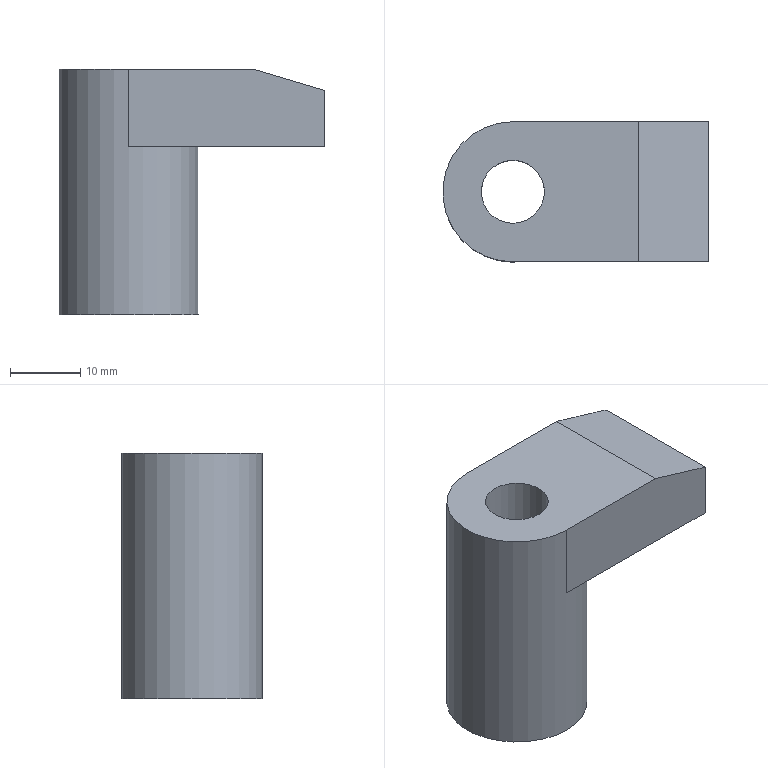Component | NX | HOOK_CLAMP_PLATE | 1 solid | 11 faces | box 38 x 20 x 35 mm | volume 11095 mm3 | plane 8 | cylinder 3 | commonest cylinder face diameters 9 x1 20 x1 14 x1
STEP:
#1=CARTESIAN_POINT('',(0.,0.,0.));
#2=DIRECTION('',(0.,0.,1.));
#3=DIRECTION('',(1.,0.,0.));
#4=AXIS2_PLACEMENT_3D('',#1,#2,#3);
#5=CARTESIAN_POINT('',(117.5,-4.5,-27.));
#6=VERTEX_POINT('',#5);
#7=CARTESIAN_POINT('',(117.5,-0.,-27.));
#8=DIRECTION('',(0.,0.,1.));
#9=DIRECTION('',(0.,-1.,0.));
#10=AXIS2_PLACEMENT_3D('',#7,#8,#9);
#11=CIRCLE('',#10,4.5);
#12=CARTESIAN_POINT('',(117.5,-0.,-62.));
#13=DIRECTION('',(0.,0.,1.));
#14=DIRECTION('',(0.,-1.,0.));
#15=AXIS2_PLACEMENT_3D('',#12,#13,#14);
#16=CYLINDRICAL_SURFACE('',#15,4.5);
#17=CARTESIAN_POINT('',(0.,35.));
#18=DIRECTION('',(1.,0.));
#19=VECTOR('',#18,1.);
#20=LINE('',#17,#19);
#21=(GEOMETRIC_REPRESENTATION_CONTEXT(2)PARAMETRIC_REPRESENTATION_CONTEXT()REPRESENTATION_CONTEXT('',''));
#22=DEFINITIONAL_REPRESENTATION('',(#20),#21);
#23=PCURVE('',#16,#22);
#24=CARTESIAN_POINT('',(117.5,-0.,-27.));
#25=DIRECTION('',(0.,0.,1.));
#26=DIRECTION('',(0.,-1.,0.));
#27=AXIS2_PLACEMENT_3D('',#24,#25,#26);
#28=PLANE('',#27);
#29=CARTESIAN_POINT('',(0.,0.));
#30=DIRECTION('',(1.,0.));
#31=AXIS2_PLACEMENT_2D('',#29,#30);
#32=CIRCLE('',#31,4.5);
#33=(GEOMETRIC_REPRESENTATION_CONTEXT(2)PARAMETRIC_REPRESENTATION_CONTEXT()REPRESENTATION_CONTEXT('',''));
#34=DEFINITIONAL_REPRESENTATION('',(#32),#33);
#35=PCURVE('',#28,#34);
#36=SURFACE_CURVE('',#11,(#23,#35),.PCURVE_S1.);
#37=EDGE_CURVE('',#6,#6,#36,.T.);
#38=ORIENTED_EDGE('',*,*,#37,.F.);
#39=CARTESIAN_POINT('',(117.5,-4.5,-42.));
#40=VERTEX_POINT('',#39);
#41=CARTESIAN_POINT('',(117.5,-4.5,-42.));
#42=CARTESIAN_POINT('',(117.5,-4.5,-27.));
#43=B_SPLINE_CURVE_WITH_KNOTS('',1,(#41,#42),.UNSPECIFIED.,.F.,.F.,(2,2),(20.,35.),.PIECEWISE_BEZIER_KNOTS.);
#44=CARTESIAN_POINT('',(0.,0.));
#45=DIRECTION('',(0.,1.));
#46=VECTOR('',#45,1.);
#47=LINE('',#44,#46);
#48=(GEOMETRIC_REPRESENTATION_CONTEXT(2)PARAMETRIC_REPRESENTATION_CONTEXT()REPRESENTATION_CONTEXT('',''));
#49=DEFINITIONAL_REPRESENTATION('',(#47),#48);
#50=PCURVE('',#16,#49);
#51=CARTESIAN_POINT('',(6.283,0.));
#52=DIRECTION('',(0.,1.));
#53=VECTOR('',#52,1.);
#54=LINE('',#51,#53);
#55=(GEOMETRIC_REPRESENTATION_CONTEXT(2)PARAMETRIC_REPRESENTATION_CONTEXT()REPRESENTATION_CONTEXT('',''));
#56=DEFINITIONAL_REPRESENTATION('',(#54),#55);
#57=PCURVE('',#16,#56);
#58=SEAM_CURVE('',#43,(#50,#57),.PCURVE_S1.);
#59=EDGE_CURVE('',#40,#6,#58,.T.);
#60=ORIENTED_EDGE('',*,*,#59,.F.);
#61=CARTESIAN_POINT('',(117.5,4.5,-42.));
#62=VERTEX_POINT('',#61);
#63=CARTESIAN_POINT('',(117.5,-0.,-42.));
#64=DIRECTION('',(0.,0.,1.));
#65=DIRECTION('',(0.,1.,0.));
#66=AXIS2_PLACEMENT_3D('',#63,#64,#65);
#67=CIRCLE('',#66,4.5);
#68=CARTESIAN_POINT('',(-3.142,20.));
#69=DIRECTION('',(1.,0.));
#70=VECTOR('',#69,1.);
#71=LINE('',#68,#70);
#72=(GEOMETRIC_REPRESENTATION_CONTEXT(2)PARAMETRIC_REPRESENTATION_CONTEXT()REPRESENTATION_CONTEXT('',''));
#73=DEFINITIONAL_REPRESENTATION('',(#71),#72);
#74=PCURVE('',#16,#73);
#75=CARTESIAN_POINT('',(117.5,-0.,-42.));
#76=DIRECTION('',(0.,0.,-1.));
#77=DIRECTION('',(0.,1.,0.));
#78=AXIS2_PLACEMENT_3D('',#75,#76,#77);
#79=PLANE('',#78);
#80=CARTESIAN_POINT('',(4.5,0.));
#81=CARTESIAN_POINT('',(4.5,-7.794));
#82=CARTESIAN_POINT('',(-2.25,-3.897));
#83=CARTESIAN_POINT('',(-9.,-0.));
#84=CARTESIAN_POINT('',(-2.25,3.897));
#85=CARTESIAN_POINT('',(4.5,7.794));
#86=CARTESIAN_POINT('',(4.5,0.));
#87=(BOUNDED_CURVE()B_SPLINE_CURVE(2,(#80,#81,#82,#83,#84,#85,#86),.UNSPECIFIED.,.T.,.F.)B_SPLINE_CURVE_WITH_KNOTS((1,2,2,2,2,1),(-2.094,0.,2.094,4.189,6.283,8.378),.UNSPECIFIED.)CURVE()GEOMETRIC_REPRESENTATION_ITEM()RATIONAL_B_SPLINE_CURVE((1.,0.5,1.,0.5,1.,0.5,1.))REPRESENTATION_ITEM(''));
#88=(GEOMETRIC_REPRESENTATION_CONTEXT(2)PARAMETRIC_REPRESENTATION_CONTEXT()REPRESENTATION_CONTEXT('',''));
#89=DEFINITIONAL_REPRESENTATION('',(#87),#88);
#90=PCURVE('',#79,#89);
#91=SURFACE_CURVE('',#67,(#74,#90),.PCURVE_S1.);
#92=EDGE_CURVE('',#40,#62,#91,.T.);
#93=ORIENTED_EDGE('',*,*,#92,.T.);
#94=CARTESIAN_POINT('',(117.5,-0.,-42.));
#95=DIRECTION('',(0.,0.,1.));
#96=DIRECTION('',(0.,1.,0.));
#97=AXIS2_PLACEMENT_3D('',#94,#95,#96);
#98=CIRCLE('',#97,4.5);
#99=CARTESIAN_POINT('',(3.142,20.));
#100=DIRECTION('',(1.,0.));
#101=VECTOR('',#100,1.);
#102=LINE('',#99,#101);
#103=(GEOMETRIC_REPRESENTATION_CONTEXT(2)PARAMETRIC_REPRESENTATION_CONTEXT()REPRESENTATION_CONTEXT('',''));
#104=DEFINITIONAL_REPRESENTATION('',(#102),#103);
#105=PCURVE('',#16,#104);
#106=CARTESIAN_POINT('',(4.5,0.));
#107=CARTESIAN_POINT('',(4.5,-7.794));
#108=CARTESIAN_POINT('',(-2.25,-3.897));
#109=CARTESIAN_POINT('',(-9.,-0.));
#110=CARTESIAN_POINT('',(-2.25,3.897));
#111=CARTESIAN_POINT('',(4.5,7.794));
#112=CARTESIAN_POINT('',(4.5,0.));
#113=(BOUNDED_CURVE()B_SPLINE_CURVE(2,(#106,#107,#108,#109,#110,#111,#112),.UNSPECIFIED.,.T.,.F.)B_SPLINE_CURVE_WITH_KNOTS((1,2,2,2,2,1),(-2.094,0.,2.094,4.189,6.283,8.378),.UNSPECIFIED.)CURVE()GEOMETRIC_REPRESENTATION_ITEM()RATIONAL_B_SPLINE_CURVE((1.,0.5,1.,0.5,1.,0.5,1.))REPRESENTATION_ITEM(''));
#114=(GEOMETRIC_REPRESENTATION_CONTEXT(2)PARAMETRIC_REPRESENTATION_CONTEXT()REPRESENTATION_CONTEXT('',''));
#115=DEFINITIONAL_REPRESENTATION('',(#113),#114);
#116=PCURVE('',#79,#115);
#117=SURFACE_CURVE('',#98,(#105,#116),.PCURVE_S1.);
#118=EDGE_CURVE('',#62,#40,#117,.T.);
#119=ORIENTED_EDGE('',*,*,#118,.T.);
#120=ORIENTED_EDGE('',*,*,#59,.T.);
#121=EDGE_LOOP('',(#38,#60,#93,#119,#120));
#122=FACE_BOUND('',#121,.F.);
#123=ADVANCED_FACE('',(#122),#16,.F.);
#124=CARTESIAN_POINT('',(117.5,10.,-38.));
#125=VERTEX_POINT('',#124);
#126=CARTESIAN_POINT('',(117.5,10.,-27.));
#127=VERTEX_POINT('',#126);
#128=CARTESIAN_POINT('',(117.5,10.,-38.));
#129=DIRECTION('',(0.,0.,1.));
#130=VECTOR('',#129,1.);
#131=LINE('',#128,#130);
#132=CARTESIAN_POINT('',(117.5,-0.,-62.));
#133=DIRECTION('',(0.,0.,1.));
#134=DIRECTION('',(0.,-1.,0.));
#135=AXIS2_PLACEMENT_3D('',#132,#133,#134);
#136=CYLINDRICAL_SURFACE('',#135,10.);
#137=CARTESIAN_POINT('',(3.142,24.));
#138=DIRECTION('',(0.,1.));
#139=VECTOR('',#138,1.);
#140=LINE('',#137,#139);
#141=(GEOMETRIC_REPRESENTATION_CONTEXT(2)PARAMETRIC_REPRESENTATION_CONTEXT()REPRESENTATION_CONTEXT('',''));
#142=DEFINITIONAL_REPRESENTATION('',(#140),#141);
#143=PCURVE('',#136,#142);
#144=CARTESIAN_POINT('',(145.5,10.,-38.));
#145=DIRECTION('',(0.,1.,0.));
#146=DIRECTION('',(0.,0.,1.));
#147=AXIS2_PLACEMENT_3D('',#144,#145,#146);
#148=PLANE('',#147);
#149=CARTESIAN_POINT('',(0.,-28.));
#150=DIRECTION('',(1.,0.));
#151=VECTOR('',#150,1.);
#152=LINE('',#149,#151);
#153=(GEOMETRIC_REPRESENTATION_CONTEXT(2)PARAMETRIC_REPRESENTATION_CONTEXT()REPRESENTATION_CONTEXT('',''));
#154=DEFINITIONAL_REPRESENTATION('',(#152),#153);
#155=PCURVE('',#148,#154);
#156=SURFACE_CURVE('',#131,(#143,#155),.PCURVE_S1.);
#157=EDGE_CURVE('',#125,#127,#156,.T.);
#158=ORIENTED_EDGE('',*,*,#157,.F.);
#159=CARTESIAN_POINT('',(117.5,-10.,-38.));
#160=VERTEX_POINT('',#159);
#161=CARTESIAN_POINT('',(117.5,-0.,-38.));
#162=DIRECTION('',(0.,0.,-1.));
#163=DIRECTION('',(0.,-1.,0.));
#164=AXIS2_PLACEMENT_3D('',#161,#162,#163);
#165=CIRCLE('',#164,10.);
#166=CARTESIAN_POINT('',(6.283,24.));
#167=DIRECTION('',(-1.,0.));
#168=VECTOR('',#167,1.);
#169=LINE('',#166,#168);
#170=(GEOMETRIC_REPRESENTATION_CONTEXT(2)PARAMETRIC_REPRESENTATION_CONTEXT()REPRESENTATION_CONTEXT('',''));
#171=DEFINITIONAL_REPRESENTATION('',(#169),#170);
#172=PCURVE('',#136,#171);
#173=CARTESIAN_POINT('',(117.5,-0.,-38.));
#174=DIRECTION('',(0.,0.,-1.));
#175=DIRECTION('',(0.,1.,0.));
#176=AXIS2_PLACEMENT_3D('',#173,#174,#175);
#177=PLANE('',#176);
#178=CARTESIAN_POINT('',(0.,0.));
#179=DIRECTION('',(-1.,0.));
#180=AXIS2_PLACEMENT_2D('',#178,#179);
#181=CIRCLE('',#180,10.);
#182=(GEOMETRIC_REPRESENTATION_CONTEXT(2)PARAMETRIC_REPRESENTATION_CONTEXT()REPRESENTATION_CONTEXT('',''));
#183=DEFINITIONAL_REPRESENTATION('',(#181),#182);
#184=PCURVE('',#177,#183);
#185=SURFACE_CURVE('',#165,(#172,#184),.PCURVE_S1.);
#186=EDGE_CURVE('',#125,#160,#185,.T.);
#187=ORIENTED_EDGE('',*,*,#186,.T.);
#188=CARTESIAN_POINT('',(117.5,-10.,-62.));
#189=VERTEX_POINT('',#188);
#190=CARTESIAN_POINT('',(117.5,-10.,-62.));
#191=CARTESIAN_POINT('',(117.5,-10.,-38.));
#192=B_SPLINE_CURVE_WITH_KNOTS('',1,(#190,#191),.UNSPECIFIED.,.F.,.F.,(2,2),(0.,24.),.PIECEWISE_BEZIER_KNOTS.);
#193=CARTESIAN_POINT('',(0.,0.));
#194=DIRECTION('',(0.,1.));
#195=VECTOR('',#194,1.);
#196=LINE('',#193,#195);
#197=(GEOMETRIC_REPRESENTATION_CONTEXT(2)PARAMETRIC_REPRESENTATION_CONTEXT()REPRESENTATION_CONTEXT('',''));
#198=DEFINITIONAL_REPRESENTATION('',(#196),#197);
#199=PCURVE('',#136,#198);
#200=CARTESIAN_POINT('',(6.283,0.));
#201=DIRECTION('',(0.,1.));
#202=VECTOR('',#201,1.);
#203=LINE('',#200,#202);
#204=(GEOMETRIC_REPRESENTATION_CONTEXT(2)PARAMETRIC_REPRESENTATION_CONTEXT()REPRESENTATION_CONTEXT('',''));
#205=DEFINITIONAL_REPRESENTATION('',(#203),#204);
#206=PCURVE('',#136,#205);
#207=SEAM_CURVE('',#192,(#199,#206),.PCURVE_S1.);
#208=EDGE_CURVE('',#189,#160,#207,.T.);
#209=ORIENTED_EDGE('',*,*,#208,.F.);
#210=CARTESIAN_POINT('',(117.5,-0.,-62.));
#211=DIRECTION('',(0.,0.,1.));
#212=DIRECTION('',(0.,-1.,0.));
#213=AXIS2_PLACEMENT_3D('',#210,#211,#212);
#214=CIRCLE('',#213,10.);
#215=CARTESIAN_POINT('',(0.,0.));
#216=DIRECTION('',(1.,0.));
#217=VECTOR('',#216,1.);
#218=LINE('',#215,#217);
#219=(GEOMETRIC_REPRESENTATION_CONTEXT(2)PARAMETRIC_REPRESENTATION_CONTEXT()REPRESENTATION_CONTEXT('',''));
#220=DEFINITIONAL_REPRESENTATION('',(#218),#219);
#221=PCURVE('',#136,#220);
#222=CARTESIAN_POINT('',(117.5,-0.,-62.));
#223=DIRECTION('',(0.,0.,1.));
#224=DIRECTION('',(0.,-1.,0.));
#225=AXIS2_PLACEMENT_3D('',#222,#223,#224);
#226=PLANE('',#225);
#227=CARTESIAN_POINT('',(0.,0.));
#228=DIRECTION('',(1.,0.));
#229=AXIS2_PLACEMENT_2D('',#227,#228);
#230=CIRCLE('',#229,10.);
#231=(GEOMETRIC_REPRESENTATION_CONTEXT(2)PARAMETRIC_REPRESENTATION_CONTEXT()REPRESENTATION_CONTEXT('',''));
#232=DEFINITIONAL_REPRESENTATION('',(#230),#231);
#233=PCURVE('',#226,#232);
#234=SURFACE_CURVE('',#214,(#221,#233),.PCURVE_S1.);
#235=EDGE_CURVE('',#189,#189,#234,.T.);
#236=ORIENTED_EDGE('',*,*,#235,.T.);
#237=ORIENTED_EDGE('',*,*,#208,.T.);
#238=CARTESIAN_POINT('',(117.5,-10.,-27.));
#239=VERTEX_POINT('',#238);
#240=CARTESIAN_POINT('',(117.5,-10.,-38.));
#241=DIRECTION('',(0.,0.,1.));
#242=VECTOR('',#241,1.);
#243=LINE('',#240,#242);
#244=CARTESIAN_POINT('',(6.283,24.));
#245=DIRECTION('',(0.,1.));
#246=VECTOR('',#245,1.);
#247=LINE('',#244,#246);
#248=(GEOMETRIC_REPRESENTATION_CONTEXT(2)PARAMETRIC_REPRESENTATION_CONTEXT()REPRESENTATION_CONTEXT('',''));
#249=DEFINITIONAL_REPRESENTATION('',(#247),#248);
#250=PCURVE('',#136,#249);
#251=CARTESIAN_POINT('',(117.5,-10.,-38.));
#252=DIRECTION('',(0.,-1.,0.));
#253=DIRECTION('',(0.,0.,-1.));
#254=AXIS2_PLACEMENT_3D('',#251,#252,#253);
#255=PLANE('',#254);
#256=CARTESIAN_POINT('',(0.,0.));
#257=DIRECTION('',(-1.,0.));
#258=VECTOR('',#257,1.);
#259=LINE('',#256,#258);
#260=(GEOMETRIC_REPRESENTATION_CONTEXT(2)PARAMETRIC_REPRESENTATION_CONTEXT()REPRESENTATION_CONTEXT('',''));
#261=DEFINITIONAL_REPRESENTATION('',(#259),#260);
#262=PCURVE('',#255,#261);
#263=SURFACE_CURVE('',#243,(#250,#262),.PCURVE_S1.);
#264=EDGE_CURVE('',#160,#239,#263,.T.);
#265=ORIENTED_EDGE('',*,*,#264,.T.);
#266=CARTESIAN_POINT('',(117.5,-0.,-27.));
#267=DIRECTION('',(0.,0.,1.));
#268=DIRECTION('',(0.,-1.,0.));
#269=AXIS2_PLACEMENT_3D('',#266,#267,#268);
#270=CIRCLE('',#269,10.);
#271=CARTESIAN_POINT('',(0.,35.));
#272=DIRECTION('',(1.,0.));
#273=VECTOR('',#272,1.);
#274=LINE('',#271,#273);
#275=(GEOMETRIC_REPRESENTATION_CONTEXT(2)PARAMETRIC_REPRESENTATION_CONTEXT()REPRESENTATION_CONTEXT('',''));
#276=DEFINITIONAL_REPRESENTATION('',(#274),#275);
#277=PCURVE('',#136,#276);
#278=CARTESIAN_POINT('',(0.,0.));
#279=DIRECTION('',(1.,0.));
#280=AXIS2_PLACEMENT_2D('',#278,#279);
#281=CIRCLE('',#280,10.);
#282=(GEOMETRIC_REPRESENTATION_CONTEXT(2)PARAMETRIC_REPRESENTATION_CONTEXT()REPRESENTATION_CONTEXT('',''));
#283=DEFINITIONAL_REPRESENTATION('',(#281),#282);
#284=PCURVE('',#28,#283);
#285=SURFACE_CURVE('',#270,(#277,#284),.PCURVE_S1.);
#286=EDGE_CURVE('',#127,#239,#285,.T.);
#287=ORIENTED_EDGE('',*,*,#286,.F.);
#288=EDGE_LOOP('',(#158,#187,#209,#236,#237,#265,#287));
#289=FACE_BOUND('',#288,.T.);
#290=ADVANCED_FACE('',(#289),#136,.T.);
#291=CARTESIAN_POINT('',(117.5,-7.,-62.));
#292=VERTEX_POINT('',#291);
#293=CARTESIAN_POINT('',(117.5,-0.,-62.));
#294=DIRECTION('',(0.,0.,-1.));
#295=DIRECTION('',(0.,-1.,0.));
#296=AXIS2_PLACEMENT_3D('',#293,#294,#295);
#297=CIRCLE('',#296,7.);
#298=CARTESIAN_POINT('',(7.,0.));
#299=CARTESIAN_POINT('',(7.,-12.124));
#300=CARTESIAN_POINT('',(-3.5,-6.062));
#301=CARTESIAN_POINT('',(-14.,-0.));
#302=CARTESIAN_POINT('',(-3.5,6.062));
#303=CARTESIAN_POINT('',(7.,12.124));
#304=CARTESIAN_POINT('',(7.,0.));
#305=(BOUNDED_CURVE()B_SPLINE_CURVE(2,(#298,#299,#300,#301,#302,#303,#304),.UNSPECIFIED.,.T.,.F.)B_SPLINE_CURVE_WITH_KNOTS((1,2,2,2,2,1),(-2.094,0.,2.094,4.189,6.283,8.378),.UNSPECIFIED.)CURVE()GEOMETRIC_REPRESENTATION_ITEM()RATIONAL_B_SPLINE_CURVE((1.,0.5,1.,0.5,1.,0.5,1.))REPRESENTATION_ITEM(''));
#306=(GEOMETRIC_REPRESENTATION_CONTEXT(2)PARAMETRIC_REPRESENTATION_CONTEXT()REPRESENTATION_CONTEXT('',''));
#307=DEFINITIONAL_REPRESENTATION('',(#305),#306);
#308=PCURVE('',#226,#307);
#309=CARTESIAN_POINT('',(117.5,-0.,-42.));
#310=DIRECTION('',(0.,0.,-1.));
#311=DIRECTION('',(0.,1.,0.));
#312=AXIS2_PLACEMENT_3D('',#309,#310,#311);
#313=CYLINDRICAL_SURFACE('',#312,7.);
#314=CARTESIAN_POINT('',(3.142,20.));
#315=DIRECTION('',(1.,0.));
#316=VECTOR('',#315,1.);
#317=LINE('',#314,#316);
#318=(GEOMETRIC_REPRESENTATION_CONTEXT(2)PARAMETRIC_REPRESENTATION_CONTEXT()REPRESENTATION_CONTEXT('',''));
#319=DEFINITIONAL_REPRESENTATION('',(#317),#318);
#320=PCURVE('',#313,#319);
#321=SURFACE_CURVE('',#297,(#308,#320),.PCURVE_S1.);
#322=EDGE_CURVE('',#292,#292,#321,.T.);
#323=ORIENTED_EDGE('',*,*,#322,.F.);
#324=EDGE_LOOP('',(#323));
#325=FACE_BOUND('',#324,.T.);
#326=ORIENTED_EDGE('',*,*,#235,.F.);
#327=EDGE_LOOP('',(#326));
#328=FACE_BOUND('',#327,.T.);
#329=ADVANCED_FACE('',(#325,#328),#226,.F.);
#330=CARTESIAN_POINT('',(135.5,-10.,-27.));
#331=VERTEX_POINT('',#330);
#332=CARTESIAN_POINT('',(117.5,-10.,-27.));
#333=DIRECTION('',(1.,0.,0.));
#334=VECTOR('',#333,1.);
#335=LINE('',#332,#334);
#336=CARTESIAN_POINT('',(10.,0.));
#337=DIRECTION('',(0.,1.));
#338=VECTOR('',#337,1.);
#339=LINE('',#336,#338);
#340=(GEOMETRIC_REPRESENTATION_CONTEXT(2)PARAMETRIC_REPRESENTATION_CONTEXT()REPRESENTATION_CONTEXT('',''));
#341=DEFINITIONAL_REPRESENTATION('',(#339),#340);
#342=PCURVE('',#28,#341);
#343=CARTESIAN_POINT('',(-11.,0.));
#344=DIRECTION('',(0.,1.));
#345=VECTOR('',#344,1.);
#346=LINE('',#343,#345);
#347=(GEOMETRIC_REPRESENTATION_CONTEXT(2)PARAMETRIC_REPRESENTATION_CONTEXT()REPRESENTATION_CONTEXT('',''));
#348=DEFINITIONAL_REPRESENTATION('',(#346),#347);
#349=PCURVE('',#255,#348);
#350=SURFACE_CURVE('',#335,(#342,#349),.PCURVE_S1.);
#351=EDGE_CURVE('',#239,#331,#350,.T.);
#352=ORIENTED_EDGE('',*,*,#351,.T.);
#353=CARTESIAN_POINT('',(135.5,10.,-27.));
#354=VERTEX_POINT('',#353);
#355=CARTESIAN_POINT('',(135.5,-0.,-27.));
#356=DIRECTION('',(0.,1.,0.));
#357=VECTOR('',#356,1.);
#358=LINE('',#355,#357);
#359=CARTESIAN_POINT('',(0.,18.));
#360=DIRECTION('',(-1.,0.));
#361=VECTOR('',#360,1.);
#362=LINE('',#359,#361);
#363=(GEOMETRIC_REPRESENTATION_CONTEXT(2)PARAMETRIC_REPRESENTATION_CONTEXT()REPRESENTATION_CONTEXT('',''));
#364=DEFINITIONAL_REPRESENTATION('',(#362),#363);
#365=PCURVE('',#28,#364);
#366=CARTESIAN_POINT('',(135.5,-0.,-27.));
#367=DIRECTION('',(-0.2873,0.,-0.9578));
#368=DIRECTION('',(0.,1.,0.));
#369=AXIS2_PLACEMENT_3D('',#366,#367,#368);
#370=PLANE('',#369);
#371=CARTESIAN_POINT('',(0.,0.));
#372=DIRECTION('',(1.,0.));
#373=VECTOR('',#372,1.);
#374=LINE('',#371,#373);
#375=(GEOMETRIC_REPRESENTATION_CONTEXT(2)PARAMETRIC_REPRESENTATION_CONTEXT()REPRESENTATION_CONTEXT('',''));
#376=DEFINITIONAL_REPRESENTATION('',(#374),#375);
#377=PCURVE('',#370,#376);
#378=SURFACE_CURVE('',#358,(#365,#377),.PCURVE_S1.);
#379=EDGE_CURVE('',#331,#354,#378,.T.);
#380=ORIENTED_EDGE('',*,*,#379,.T.);
#381=CARTESIAN_POINT('',(145.5,10.,-27.));
#382=DIRECTION('',(-1.,0.,0.));
#383=VECTOR('',#382,1.);
#384=LINE('',#381,#383);
#385=CARTESIAN_POINT('',(-10.,28.));
#386=DIRECTION('',(0.,-1.));
#387=VECTOR('',#386,1.);
#388=LINE('',#385,#387);
#389=(GEOMETRIC_REPRESENTATION_CONTEXT(2)PARAMETRIC_REPRESENTATION_CONTEXT()REPRESENTATION_CONTEXT('',''));
#390=DEFINITIONAL_REPRESENTATION('',(#388),#389);
#391=PCURVE('',#28,#390);
#392=CARTESIAN_POINT('',(11.,0.));
#393=DIRECTION('',(0.,-1.));
#394=VECTOR('',#393,1.);
#395=LINE('',#392,#394);
#396=(GEOMETRIC_REPRESENTATION_CONTEXT(2)PARAMETRIC_REPRESENTATION_CONTEXT()REPRESENTATION_CONTEXT('',''));
#397=DEFINITIONAL_REPRESENTATION('',(#395),#396);
#398=PCURVE('',#148,#397);
#399=SURFACE_CURVE('',#384,(#391,#398),.PCURVE_S1.);
#400=EDGE_CURVE('',#354,#127,#399,.T.);
#401=ORIENTED_EDGE('',*,*,#400,.T.);
#402=ORIENTED_EDGE('',*,*,#286,.T.);
#403=EDGE_LOOP('',(#352,#380,#401,#402));
#404=FACE_BOUND('',#403,.T.);
#405=ORIENTED_EDGE('',*,*,#37,.F.);
#406=EDGE_LOOP('',(#405));
#407=FACE_BOUND('',#406,.T.);
#408=ADVANCED_FACE('',(#404,#407),#28,.T.);
#409=ORIENTED_EDGE('',*,*,#400,.F.);
#410=CARTESIAN_POINT('',(145.5,10.,-30.));
#411=VERTEX_POINT('',#410);
#412=CARTESIAN_POINT('',(147.702,10.,-30.661));
#413=DIRECTION('',(0.9578,0.,-0.2873));
#414=VECTOR('',#413,1.);
#415=LINE('',#412,#414);
#416=CARTESIAN_POINT('',(7.339,2.202));
#417=DIRECTION('',(-0.2873,0.9578));
#418=VECTOR('',#417,1.);
#419=LINE('',#416,#418);
#420=(GEOMETRIC_REPRESENTATION_CONTEXT(2)PARAMETRIC_REPRESENTATION_CONTEXT()REPRESENTATION_CONTEXT('',''));
#421=DEFINITIONAL_REPRESENTATION('',(#419),#420);
#422=PCURVE('',#148,#421);
#423=CARTESIAN_POINT('',(10.,12.739));
#424=DIRECTION('',(0.,1.));
#425=VECTOR('',#424,1.);
#426=LINE('',#423,#425);
#427=(GEOMETRIC_REPRESENTATION_CONTEXT(2)PARAMETRIC_REPRESENTATION_CONTEXT()REPRESENTATION_CONTEXT('',''));
#428=DEFINITIONAL_REPRESENTATION('',(#426),#427);
#429=PCURVE('',#370,#428);
#430=SURFACE_CURVE('',#415,(#422,#429),.PCURVE_S1.);
#431=EDGE_CURVE('',#354,#411,#430,.T.);
#432=ORIENTED_EDGE('',*,*,#431,.T.);
#433=CARTESIAN_POINT('',(145.5,10.,-38.));
#434=VERTEX_POINT('',#433);
#435=CARTESIAN_POINT('',(145.5,10.,-38.));
#436=DIRECTION('',(0.,0.,1.));
#437=VECTOR('',#436,1.);
#438=LINE('',#435,#437);
#439=CARTESIAN_POINT('',(0.,0.));
#440=DIRECTION('',(1.,0.));
#441=VECTOR('',#440,1.);
#442=LINE('',#439,#441);
#443=(GEOMETRIC_REPRESENTATION_CONTEXT(2)PARAMETRIC_REPRESENTATION_CONTEXT()REPRESENTATION_CONTEXT('',''));
#444=DEFINITIONAL_REPRESENTATION('',(#442),#443);
#445=PCURVE('',#148,#444);
#446=CARTESIAN_POINT('',(145.5,-10.,-38.));
#447=DIRECTION('',(1.,0.,0.));
#448=DIRECTION('',(0.,0.,1.));
#449=AXIS2_PLACEMENT_3D('',#446,#447,#448);
#450=PLANE('',#449);
#451=CARTESIAN_POINT('',(0.,-20.));
#452=DIRECTION('',(1.,0.));
#453=VECTOR('',#452,1.);
#454=LINE('',#451,#453);
#455=(GEOMETRIC_REPRESENTATION_CONTEXT(2)PARAMETRIC_REPRESENTATION_CONTEXT()REPRESENTATION_CONTEXT('',''));
#456=DEFINITIONAL_REPRESENTATION('',(#454),#455);
#457=PCURVE('',#450,#456);
#458=SURFACE_CURVE('',#438,(#445,#457),.PCURVE_S1.);
#459=EDGE_CURVE('',#434,#411,#458,.T.);
#460=ORIENTED_EDGE('',*,*,#459,.F.);
#461=CARTESIAN_POINT('',(145.5,10.,-38.));
#462=DIRECTION('',(-1.,0.,0.));
#463=VECTOR('',#462,1.);
#464=LINE('',#461,#463);
#465=CARTESIAN_POINT('',(0.,0.));
#466=DIRECTION('',(0.,-1.));
#467=VECTOR('',#466,1.);
#468=LINE('',#465,#467);
#469=(GEOMETRIC_REPRESENTATION_CONTEXT(2)PARAMETRIC_REPRESENTATION_CONTEXT()REPRESENTATION_CONTEXT('',''));
#470=DEFINITIONAL_REPRESENTATION('',(#468),#469);
#471=PCURVE('',#148,#470);
#472=CARTESIAN_POINT('',(10.,28.));
#473=DIRECTION('',(0.,-1.));
#474=VECTOR('',#473,1.);
#475=LINE('',#472,#474);
#476=(GEOMETRIC_REPRESENTATION_CONTEXT(2)PARAMETRIC_REPRESENTATION_CONTEXT()REPRESENTATION_CONTEXT('',''));
#477=DEFINITIONAL_REPRESENTATION('',(#475),#476);
#478=PCURVE('',#177,#477);
#479=SURFACE_CURVE('',#464,(#471,#478),.PCURVE_S1.);
#480=EDGE_CURVE('',#434,#125,#479,.T.);
#481=ORIENTED_EDGE('',*,*,#480,.T.);
#482=ORIENTED_EDGE('',*,*,#157,.T.);
#483=EDGE_LOOP('',(#409,#432,#460,#481,#482));
#484=FACE_BOUND('',#483,.T.);
#485=ADVANCED_FACE('',(#484),#148,.T.);
#486=CARTESIAN_POINT('',(145.5,-10.,-38.));
#487=VERTEX_POINT('',#486);
#488=CARTESIAN_POINT('',(145.5,-10.,-30.));
#489=VERTEX_POINT('',#488);
#490=CARTESIAN_POINT('',(145.5,-10.,-38.));
#491=DIRECTION('',(0.,0.,1.));
#492=VECTOR('',#491,1.);
#493=LINE('',#490,#492);
#494=CARTESIAN_POINT('',(0.,28.));
#495=DIRECTION('',(-1.,0.));
#496=VECTOR('',#495,1.);
#497=LINE('',#494,#496);
#498=(GEOMETRIC_REPRESENTATION_CONTEXT(2)PARAMETRIC_REPRESENTATION_CONTEXT()REPRESENTATION_CONTEXT('',''));
#499=DEFINITIONAL_REPRESENTATION('',(#497),#498);
#500=PCURVE('',#255,#499);
#501=CARTESIAN_POINT('',(0.,0.));
#502=DIRECTION('',(1.,0.));
#503=VECTOR('',#502,1.);
#504=LINE('',#501,#503);
#505=(GEOMETRIC_REPRESENTATION_CONTEXT(2)PARAMETRIC_REPRESENTATION_CONTEXT()REPRESENTATION_CONTEXT('',''));
#506=DEFINITIONAL_REPRESENTATION('',(#504),#505);
#507=PCURVE('',#450,#506);
#508=SURFACE_CURVE('',#493,(#500,#507),.PCURVE_S1.);
#509=EDGE_CURVE('',#487,#489,#508,.T.);
#510=ORIENTED_EDGE('',*,*,#509,.T.);
#511=CARTESIAN_POINT('',(122.014,-10.,-22.954));
#512=DIRECTION('',(-0.9578,0.,0.2873));
#513=VECTOR('',#512,1.);
#514=LINE('',#511,#513);
#515=CARTESIAN_POINT('',(-15.046,4.514));
#516=DIRECTION('',(-0.2873,-0.9578));
#517=VECTOR('',#516,1.);
#518=LINE('',#515,#517);
#519=(GEOMETRIC_REPRESENTATION_CONTEXT(2)PARAMETRIC_REPRESENTATION_CONTEXT()REPRESENTATION_CONTEXT('',''));
#520=DEFINITIONAL_REPRESENTATION('',(#518),#519);
#521=PCURVE('',#255,#520);
#522=CARTESIAN_POINT('',(-10.,-14.08));
#523=DIRECTION('',(0.,-1.));
#524=VECTOR('',#523,1.);
#525=LINE('',#522,#524);
#526=(GEOMETRIC_REPRESENTATION_CONTEXT(2)PARAMETRIC_REPRESENTATION_CONTEXT()REPRESENTATION_CONTEXT('',''));
#527=DEFINITIONAL_REPRESENTATION('',(#525),#526);
#528=PCURVE('',#370,#527);
#529=SURFACE_CURVE('',#514,(#521,#528),.PCURVE_S1.);
#530=EDGE_CURVE('',#489,#331,#529,.T.);
#531=ORIENTED_EDGE('',*,*,#530,.T.);
#532=ORIENTED_EDGE('',*,*,#351,.F.);
#533=ORIENTED_EDGE('',*,*,#264,.F.);
#534=CARTESIAN_POINT('',(117.5,-10.,-38.));
#535=DIRECTION('',(1.,0.,0.));
#536=VECTOR('',#535,1.);
#537=LINE('',#534,#536);
#538=CARTESIAN_POINT('',(0.,0.));
#539=DIRECTION('',(0.,1.));
#540=VECTOR('',#539,1.);
#541=LINE('',#538,#540);
#542=(GEOMETRIC_REPRESENTATION_CONTEXT(2)PARAMETRIC_REPRESENTATION_CONTEXT()REPRESENTATION_CONTEXT('',''));
#543=DEFINITIONAL_REPRESENTATION('',(#541),#542);
#544=PCURVE('',#255,#543);
#545=CARTESIAN_POINT('',(-10.,0.));
#546=DIRECTION('',(0.,1.));
#547=VECTOR('',#546,1.);
#548=LINE('',#545,#547);
#549=(GEOMETRIC_REPRESENTATION_CONTEXT(2)PARAMETRIC_REPRESENTATION_CONTEXT()REPRESENTATION_CONTEXT('',''));
#550=DEFINITIONAL_REPRESENTATION('',(#548),#549);
#551=PCURVE('',#177,#550);
#552=SURFACE_CURVE('',#537,(#544,#551),.PCURVE_S1.);
#553=EDGE_CURVE('',#160,#487,#552,.T.);
#554=ORIENTED_EDGE('',*,*,#553,.T.);
#555=EDGE_LOOP('',(#510,#531,#532,#533,#554));
#556=FACE_BOUND('',#555,.T.);
#557=ADVANCED_FACE('',(#556),#255,.T.);
#558=ORIENTED_EDGE('',*,*,#459,.T.);
#559=CARTESIAN_POINT('',(145.5,-10.,-30.));
#560=DIRECTION('',(0.,-1.,0.));
#561=VECTOR('',#560,1.);
#562=LINE('',#559,#561);
#563=CARTESIAN_POINT('',(8.,0.));
#564=DIRECTION('',(0.,1.));
#565=VECTOR('',#564,1.);
#566=LINE('',#563,#565);
#567=(GEOMETRIC_REPRESENTATION_CONTEXT(2)PARAMETRIC_REPRESENTATION_CONTEXT()REPRESENTATION_CONTEXT('',''));
#568=DEFINITIONAL_REPRESENTATION('',(#566),#567);
#569=PCURVE('',#450,#568);
#570=CARTESIAN_POINT('',(-10.,10.44));
#571=DIRECTION('',(-1.,0.));
#572=VECTOR('',#571,1.);
#573=LINE('',#570,#572);
#574=(GEOMETRIC_REPRESENTATION_CONTEXT(2)PARAMETRIC_REPRESENTATION_CONTEXT()REPRESENTATION_CONTEXT('',''));
#575=DEFINITIONAL_REPRESENTATION('',(#573),#574);
#576=PCURVE('',#370,#575);
#577=SURFACE_CURVE('',#562,(#569,#576),.PCURVE_S1.);
#578=EDGE_CURVE('',#411,#489,#577,.T.);
#579=ORIENTED_EDGE('',*,*,#578,.T.);
#580=ORIENTED_EDGE('',*,*,#509,.F.);
#581=CARTESIAN_POINT('',(145.5,-10.,-38.));
#582=DIRECTION('',(0.,1.,0.));
#583=VECTOR('',#582,1.);
#584=LINE('',#581,#583);
#585=CARTESIAN_POINT('',(0.,0.));
#586=DIRECTION('',(0.,-1.));
#587=VECTOR('',#586,1.);
#588=LINE('',#585,#587);
#589=(GEOMETRIC_REPRESENTATION_CONTEXT(2)PARAMETRIC_REPRESENTATION_CONTEXT()REPRESENTATION_CONTEXT('',''));
#590=DEFINITIONAL_REPRESENTATION('',(#588),#589);
#591=PCURVE('',#450,#590);
#592=CARTESIAN_POINT('',(-10.,28.));
#593=DIRECTION('',(1.,0.));
#594=VECTOR('',#593,1.);
#595=LINE('',#592,#594);
#596=(GEOMETRIC_REPRESENTATION_CONTEXT(2)PARAMETRIC_REPRESENTATION_CONTEXT()REPRESENTATION_CONTEXT('',''));
#597=DEFINITIONAL_REPRESENTATION('',(#595),#596);
#598=PCURVE('',#177,#597);
#599=SURFACE_CURVE('',#584,(#591,#598),.PCURVE_S1.);
#600=EDGE_CURVE('',#487,#434,#599,.T.);
#601=ORIENTED_EDGE('',*,*,#600,.T.);
#602=EDGE_LOOP('',(#558,#579,#580,#601));
#603=FACE_BOUND('',#602,.T.);
#604=ADVANCED_FACE('',(#603),#450,.T.);
#605=ORIENTED_EDGE('',*,*,#480,.F.);
#606=ORIENTED_EDGE('',*,*,#600,.F.);
#607=ORIENTED_EDGE('',*,*,#553,.F.);
#608=ORIENTED_EDGE('',*,*,#186,.F.);
#609=EDGE_LOOP('',(#605,#606,#607,#608));
#610=FACE_BOUND('',#609,.T.);
#611=ADVANCED_FACE('',(#610),#177,.T.);
#612=ORIENTED_EDGE('',*,*,#530,.F.);
#613=ORIENTED_EDGE('',*,*,#578,.F.);
#614=ORIENTED_EDGE('',*,*,#431,.F.);
#615=ORIENTED_EDGE('',*,*,#379,.F.);
#616=EDGE_LOOP('',(#612,#613,#614,#615));
#617=FACE_BOUND('',#616,.T.);
#618=ADVANCED_FACE('',(#617),#370,.F.);
#619=CARTESIAN_POINT('',(117.5,-7.,-42.));
#620=VERTEX_POINT('',#619);
#621=CARTESIAN_POINT('',(117.5,-0.,-42.));
#622=DIRECTION('',(0.,0.,1.));
#623=DIRECTION('',(0.,-1.,0.));
#624=AXIS2_PLACEMENT_3D('',#621,#622,#623);
#625=CIRCLE('',#624,7.);
#626=CARTESIAN_POINT('',(-7.,0.));
#627=CARTESIAN_POINT('',(-7.,12.124));
#628=CARTESIAN_POINT('',(3.5,6.062));
#629=CARTESIAN_POINT('',(14.,0.));
#630=CARTESIAN_POINT('',(3.5,-6.062));
#631=CARTESIAN_POINT('',(-7.,-12.124));
#632=CARTESIAN_POINT('',(-7.,0.));
#633=(BOUNDED_CURVE()B_SPLINE_CURVE(2,(#626,#627,#628,#629,#630,#631,#632),.UNSPECIFIED.,.T.,.F.)B_SPLINE_CURVE_WITH_KNOTS((1,2,2,2,2,1),(-2.094,0.,2.094,4.189,6.283,8.378),.UNSPECIFIED.)CURVE()GEOMETRIC_REPRESENTATION_ITEM()RATIONAL_B_SPLINE_CURVE((1.,0.5,1.,0.5,1.,0.5,1.))REPRESENTATION_ITEM(''));
#634=(GEOMETRIC_REPRESENTATION_CONTEXT(2)PARAMETRIC_REPRESENTATION_CONTEXT()REPRESENTATION_CONTEXT('',''));
#635=DEFINITIONAL_REPRESENTATION('',(#633),#634);
#636=PCURVE('',#79,#635);
#637=CARTESIAN_POINT('',(9.425,0.));
#638=DIRECTION('',(-1.,0.));
#639=VECTOR('',#638,1.);
#640=LINE('',#637,#639);
#641=(GEOMETRIC_REPRESENTATION_CONTEXT(2)PARAMETRIC_REPRESENTATION_CONTEXT()REPRESENTATION_CONTEXT('',''));
#642=DEFINITIONAL_REPRESENTATION('',(#640),#641);
#643=PCURVE('',#313,#642);
#644=SURFACE_CURVE('',#625,(#636,#643),.PCURVE_S1.);
#645=EDGE_CURVE('',#620,#620,#644,.T.);
#646=ORIENTED_EDGE('',*,*,#645,.F.);
#647=EDGE_LOOP('',(#646));
#648=FACE_BOUND('',#647,.T.);
#649=ORIENTED_EDGE('',*,*,#118,.T.);
#650=ORIENTED_EDGE('',*,*,#92,.T.);
#651=EDGE_LOOP('',(#649,#650));
#652=FACE_BOUND('',#651,.T.);
#653=ADVANCED_FACE('',(#648,#652),#79,.T.);
#654=ORIENTED_EDGE('',*,*,#645,.F.);
#655=CARTESIAN_POINT('',(117.5,-7.,-42.));
#656=CARTESIAN_POINT('',(117.5,-7.,-62.));
#657=B_SPLINE_CURVE_WITH_KNOTS('',1,(#655,#656),.UNSPECIFIED.,.F.,.F.,(2,2),(0.,20.),.PIECEWISE_BEZIER_KNOTS.);
#658=CARTESIAN_POINT('',(9.425,0.));
#659=DIRECTION('',(0.,1.));
#660=VECTOR('',#659,1.);
#661=LINE('',#658,#660);
#662=(GEOMETRIC_REPRESENTATION_CONTEXT(2)PARAMETRIC_REPRESENTATION_CONTEXT()REPRESENTATION_CONTEXT('',''));
#663=DEFINITIONAL_REPRESENTATION('',(#661),#662);
#664=PCURVE('',#313,#663);
#665=CARTESIAN_POINT('',(3.142,0.));
#666=DIRECTION('',(0.,1.));
#667=VECTOR('',#666,1.);
#668=LINE('',#665,#667);
#669=(GEOMETRIC_REPRESENTATION_CONTEXT(2)PARAMETRIC_REPRESENTATION_CONTEXT()REPRESENTATION_CONTEXT('',''));
#670=DEFINITIONAL_REPRESENTATION('',(#668),#669);
#671=PCURVE('',#313,#670);
#672=SEAM_CURVE('',#657,(#664,#671),.PCURVE_S1.);
#673=EDGE_CURVE('',#620,#292,#672,.T.);
#674=ORIENTED_EDGE('',*,*,#673,.T.);
#675=ORIENTED_EDGE('',*,*,#322,.F.);
#676=ORIENTED_EDGE('',*,*,#673,.F.);
#677=EDGE_LOOP('',(#654,#674,#675,#676));
#678=FACE_BOUND('',#677,.F.);
#679=ADVANCED_FACE('',(#678),#313,.F.);
#680=CLOSED_SHELL('',(#123,#290,#329,#408,#485,#557,#604,#611,#618,#653,#679));
#681=MANIFOLD_SOLID_BREP('',#680);
#682=(LENGTH_UNIT()NAMED_UNIT(*)SI_UNIT(.MILLI.,.METRE.));
#683=UNCERTAINTY_MEASURE_WITH_UNIT(LENGTH_MEASURE(0.000002),#682,'','');
#684=(NAMED_UNIT(*)PLANE_ANGLE_UNIT()SI_UNIT($,.RADIAN.));
#685=(NAMED_UNIT(*)SI_UNIT($,.STERADIAN.)SOLID_ANGLE_UNIT());
#686=(GEOMETRIC_REPRESENTATION_CONTEXT(3)GLOBAL_UNCERTAINTY_ASSIGNED_CONTEXT((#683))GLOBAL_UNIT_ASSIGNED_CONTEXT((#682,#684,#685))REPRESENTATION_CONTEXT('',''));
#687=ADVANCED_BREP_SHAPE_REPRESENTATION('',(#4,#681),#686);